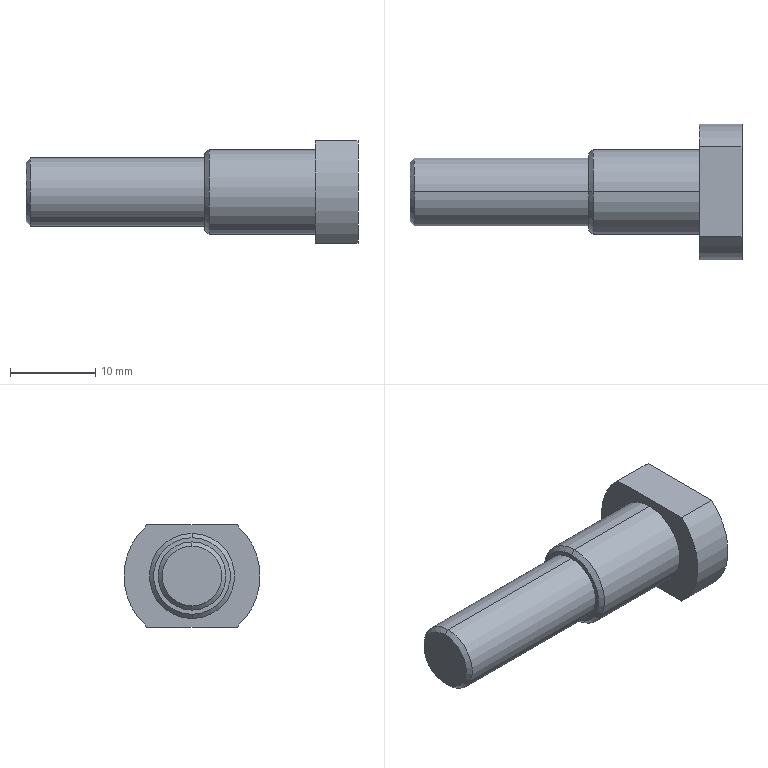Component | SolidWorks | ZTDJ-L-400-04-16-MaterialPortBagClamp-Axis4-2 | 1 solid | 16 faces | box 39 x 16 x 12 mm | volume 2930 mm3 | cylinder 6 | plane 6 | cone 4 | commonest cylinder face diameters 8 x2 10 x2 16 x2 | material 1023 Carbon Steel Sheet (SS)
STEP:
#1=COLOUR_RGB('',0.7922,0.8196,0.9333);
#2=FILL_AREA_STYLE_COLOUR('',#1);
#3=FILL_AREA_STYLE('',(#2));
#4=SURFACE_STYLE_FILL_AREA(#3);
#5=SURFACE_SIDE_STYLE('',(#4));
#6=SURFACE_STYLE_USAGE(.BOTH.,#5);
#7=PRESENTATION_STYLE_ASSIGNMENT((#6));
#8=CARTESIAN_POINT('',(2.365,-0.401,10.492));
#9=VERTEX_POINT('',#8);
#10=CARTESIAN_POINT('',(2.365,-0.401,10.217));
#11=VERTEX_POINT('',#10);
#12=CARTESIAN_POINT('',(2.365,-0.401,10.354));
#13=DIRECTION('',(-1.,0.,0.));
#14=DIRECTION('',(0.,0.,1.));
#15=AXIS2_PLACEMENT_3D('',#12,#13,#14);
#16=CIRCLE('',#15,0.1378);
#17=EDGE_CURVE('',#9,#11,#16,.T.);
#18=ORIENTED_EDGE('',*,*,#17,.F.);
#19=CARTESIAN_POINT('',(2.384,-0.401,10.512));
#20=VERTEX_POINT('',#19);
#21=CARTESIAN_POINT('',(2.365,-0.401,10.492));
#22=DIRECTION('',(0.7071,0.,0.7071));
#23=VECTOR('',#22,39.37);
#24=LINE('',#21,#23);
#25=EDGE_CURVE('',#9,#20,#24,.T.);
#26=ORIENTED_EDGE('',*,*,#25,.T.);
#27=CARTESIAN_POINT('',(2.384,-0.401,10.197));
#28=VERTEX_POINT('',#27);
#29=CARTESIAN_POINT('',(2.384,-0.401,10.354));
#30=DIRECTION('',(1.,0.,0.));
#31=DIRECTION('',(0.,0.,1.));
#32=AXIS2_PLACEMENT_3D('',#29,#30,#31);
#33=CIRCLE('',#32,0.1575);
#34=EDGE_CURVE('',#28,#20,#33,.T.);
#35=ORIENTED_EDGE('',*,*,#34,.F.);
#36=CARTESIAN_POINT('',(2.365,-0.401,10.217));
#37=DIRECTION('',(0.7071,0.,-0.7071));
#38=VECTOR('',#37,39.37);
#39=LINE('',#36,#38);
#40=EDGE_CURVE('',#11,#28,#39,.T.);
#41=ORIENTED_EDGE('',*,*,#40,.F.);
#42=EDGE_LOOP('',(#18,#26,#35,#41));
#43=FACE_OUTER_BOUND('',#42,.T.);
#44=CARTESIAN_POINT('',(2.365,-0.401,10.354));
#45=DIRECTION('',(1.,0.,0.));
#46=DIRECTION('',(0.,0.,-1.));
#47=AXIS2_PLACEMENT_3D('',#44,#45,#46);
#48=CONICAL_SURFACE('',#47,0.1378,0.7854);
#49=ADVANCED_FACE('',(#43),#48,.T.);
#50=ORIENTED_EDGE('',*,*,#34,.T.);
#51=CARTESIAN_POINT('',(3.191,-0.401,10.512));
#52=VERTEX_POINT('',#51);
#53=CARTESIAN_POINT('',(2.365,-0.401,10.512));
#54=DIRECTION('',(1.,0.,0.));
#55=VECTOR('',#54,39.37);
#56=LINE('',#53,#55);
#57=EDGE_CURVE('',#20,#52,#56,.T.);
#58=ORIENTED_EDGE('',*,*,#57,.T.);
#59=CARTESIAN_POINT('',(3.191,-0.401,10.197));
#60=VERTEX_POINT('',#59);
#61=CARTESIAN_POINT('',(3.191,-0.401,10.354));
#62=DIRECTION('',(-1.,0.,0.));
#63=DIRECTION('',(0.,0.,-1.));
#64=AXIS2_PLACEMENT_3D('',#61,#62,#63);
#65=CIRCLE('',#64,0.1575);
#66=EDGE_CURVE('',#52,#60,#65,.T.);
#67=ORIENTED_EDGE('',*,*,#66,.T.);
#68=CARTESIAN_POINT('',(2.365,-0.401,10.197));
#69=DIRECTION('',(1.,0.,0.));
#70=VECTOR('',#69,39.37);
#71=LINE('',#68,#70);
#72=EDGE_CURVE('',#28,#60,#71,.T.);
#73=ORIENTED_EDGE('',*,*,#72,.F.);
#74=EDGE_LOOP('',(#50,#58,#67,#73));
#75=FACE_OUTER_BOUND('',#74,.T.);
#76=CARTESIAN_POINT('',(2.365,-0.401,10.354));
#77=DIRECTION('',(1.,0.,0.));
#78=DIRECTION('',(0.,0.,-1.));
#79=AXIS2_PLACEMENT_3D('',#76,#77,#78);
#80=CYLINDRICAL_SURFACE('',#79,0.1575);
#81=ADVANCED_FACE('',(#75),#80,.T.);
#82=CARTESIAN_POINT('',(3.191,-0.401,10.531));
#83=VERTEX_POINT('',#82);
#84=CARTESIAN_POINT('',(3.191,-0.401,10.177));
#85=VERTEX_POINT('',#84);
#86=CARTESIAN_POINT('',(3.191,-0.401,10.354));
#87=DIRECTION('',(-1.,0.,0.));
#88=DIRECTION('',(0.,0.,-1.));
#89=AXIS2_PLACEMENT_3D('',#86,#87,#88);
#90=CIRCLE('',#89,0.1772);
#91=EDGE_CURVE('',#83,#85,#90,.T.);
#92=ORIENTED_EDGE('',*,*,#91,.F.);
#93=CARTESIAN_POINT('',(3.211,-0.401,10.551));
#94=VERTEX_POINT('',#93);
#95=CARTESIAN_POINT('',(3.211,-0.401,10.551));
#96=DIRECTION('',(0.7071,0.,0.7071));
#97=VECTOR('',#96,39.37);
#98=LINE('',#95,#97);
#99=EDGE_CURVE('',#83,#94,#98,.T.);
#100=ORIENTED_EDGE('',*,*,#99,.T.);
#101=CARTESIAN_POINT('',(3.211,-0.401,10.157));
#102=VERTEX_POINT('',#101);
#103=CARTESIAN_POINT('',(3.211,-0.401,10.354));
#104=DIRECTION('',(1.,0.,0.));
#105=DIRECTION('',(0.,0.,-1.));
#106=AXIS2_PLACEMENT_3D('',#103,#104,#105);
#107=CIRCLE('',#106,0.1969);
#108=EDGE_CURVE('',#102,#94,#107,.T.);
#109=ORIENTED_EDGE('',*,*,#108,.F.);
#110=CARTESIAN_POINT('',(3.211,-0.401,10.157));
#111=DIRECTION('',(0.7071,0.,-0.7071));
#112=VECTOR('',#111,39.37);
#113=LINE('',#110,#112);
#114=EDGE_CURVE('',#85,#102,#113,.T.);
#115=ORIENTED_EDGE('',*,*,#114,.F.);
#116=EDGE_LOOP('',(#92,#100,#109,#115));
#117=FACE_OUTER_BOUND('',#116,.T.);
#118=CARTESIAN_POINT('',(3.211,-0.401,10.354));
#119=DIRECTION('',(1.,0.,0.));
#120=DIRECTION('',(0.,0.,-1.));
#121=AXIS2_PLACEMENT_3D('',#118,#119,#120);
#122=CONICAL_SURFACE('',#121,0.1969,0.7854);
#123=ADVANCED_FACE('',(#117),#122,.T.);
#124=CARTESIAN_POINT('',(3.703,-0.401,10.157));
#125=VERTEX_POINT('',#124);
#126=CARTESIAN_POINT('',(3.703,-0.401,10.551));
#127=VERTEX_POINT('',#126);
#128=CARTESIAN_POINT('',(3.703,-0.401,10.354));
#129=DIRECTION('',(1.,0.,0.));
#130=DIRECTION('',(0.,0.,-1.));
#131=AXIS2_PLACEMENT_3D('',#128,#129,#130);
#132=CIRCLE('',#131,0.1969);
#133=EDGE_CURVE('',#125,#127,#132,.T.);
#134=ORIENTED_EDGE('',*,*,#133,.F.);
#135=CARTESIAN_POINT('',(3.703,-0.401,10.157));
#136=DIRECTION('',(-1.,0.,0.));
#137=VECTOR('',#136,39.37);
#138=LINE('',#135,#137);
#139=EDGE_CURVE('',#125,#102,#138,.T.);
#140=ORIENTED_EDGE('',*,*,#139,.T.);
#141=ORIENTED_EDGE('',*,*,#108,.T.);
#142=CARTESIAN_POINT('',(3.703,-0.401,10.551));
#143=DIRECTION('',(-1.,0.,0.));
#144=VECTOR('',#143,39.37);
#145=LINE('',#142,#144);
#146=EDGE_CURVE('',#127,#94,#145,.T.);
#147=ORIENTED_EDGE('',*,*,#146,.F.);
#148=EDGE_LOOP('',(#134,#140,#141,#147));
#149=FACE_OUTER_BOUND('',#148,.T.);
#150=CARTESIAN_POINT('',(3.703,-0.401,10.354));
#151=DIRECTION('',(-1.,0.,0.));
#152=DIRECTION('',(0.,0.,1.));
#153=AXIS2_PLACEMENT_3D('',#150,#151,#152);
#154=CYLINDRICAL_SURFACE('',#153,0.1969);
#155=ADVANCED_FACE('',(#149),#154,.T.);
#156=CARTESIAN_POINT('',(3.9,-0.6093,10.591));
#157=VERTEX_POINT('',#156);
#158=CARTESIAN_POINT('',(3.9,-0.6093,10.118));
#159=VERTEX_POINT('',#158);
#160=CARTESIAN_POINT('',(3.9,-0.401,10.354));
#161=DIRECTION('',(1.,0.,0.));
#162=DIRECTION('',(0.,0.,-1.));
#163=AXIS2_PLACEMENT_3D('',#160,#161,#162);
#164=CIRCLE('',#163,0.315);
#165=EDGE_CURVE('',#157,#159,#164,.T.);
#166=ORIENTED_EDGE('',*,*,#165,.F.);
#167=CARTESIAN_POINT('',(3.703,-0.6093,10.591));
#168=VERTEX_POINT('',#167);
#169=CARTESIAN_POINT('',(4.136,-0.6093,10.591));
#170=DIRECTION('',(-1.,0.,0.));
#171=VECTOR('',#170,39.37);
#172=LINE('',#169,#171);
#173=EDGE_CURVE('',#157,#168,#172,.T.);
#174=ORIENTED_EDGE('',*,*,#173,.T.);
#175=CARTESIAN_POINT('',(3.703,-0.6093,10.118));
#176=VERTEX_POINT('',#175);
#177=CARTESIAN_POINT('',(3.703,-0.401,10.354));
#178=DIRECTION('',(1.,0.,0.));
#179=DIRECTION('',(0.,0.,-1.));
#180=AXIS2_PLACEMENT_3D('',#177,#178,#179);
#181=CIRCLE('',#180,0.315);
#182=EDGE_CURVE('',#168,#176,#181,.T.);
#183=ORIENTED_EDGE('',*,*,#182,.T.);
#184=CARTESIAN_POINT('',(4.136,-0.6093,10.118));
#185=DIRECTION('',(-1.,0.,0.));
#186=VECTOR('',#185,39.37);
#187=LINE('',#184,#186);
#188=EDGE_CURVE('',#159,#176,#187,.T.);
#189=ORIENTED_EDGE('',*,*,#188,.F.);
#190=EDGE_LOOP('',(#166,#174,#183,#189));
#191=FACE_OUTER_BOUND('',#190,.T.);
#192=CARTESIAN_POINT('',(3.9,-0.401,10.354));
#193=DIRECTION('',(-1.,0.,0.));
#194=DIRECTION('',(0.,0.,1.));
#195=AXIS2_PLACEMENT_3D('',#192,#193,#194);
#196=CYLINDRICAL_SURFACE('',#195,0.315);
#197=ADVANCED_FACE('',(#191),#196,.T.);
#198=CARTESIAN_POINT('',(3.703,-0.401,10.354));
#199=DIRECTION('',(1.,0.,0.));
#200=DIRECTION('',(0.,0.,-1.));
#201=AXIS2_PLACEMENT_3D('',#198,#199,#200);
#202=CIRCLE('',#201,0.1969);
#203=EDGE_CURVE('',#127,#125,#202,.T.);
#204=ORIENTED_EDGE('',*,*,#203,.T.);
#205=ORIENTED_EDGE('',*,*,#133,.T.);
#206=EDGE_LOOP('',(#204,#205));
#207=FACE_BOUND('',#206,.T.);
#208=ORIENTED_EDGE('',*,*,#182,.F.);
#209=CARTESIAN_POINT('',(3.703,-0.1927,10.591));
#210=VERTEX_POINT('',#209);
#211=CARTESIAN_POINT('',(3.703,-0.401,10.591));
#212=DIRECTION('',(0.,-1.,0.));
#213=VECTOR('',#212,39.37);
#214=LINE('',#211,#213);
#215=EDGE_CURVE('',#210,#168,#214,.T.);
#216=ORIENTED_EDGE('',*,*,#215,.F.);
#217=CARTESIAN_POINT('',(3.703,-0.1927,10.118));
#218=VERTEX_POINT('',#217);
#219=CARTESIAN_POINT('',(3.703,-0.401,10.354));
#220=DIRECTION('',(1.,0.,0.));
#221=DIRECTION('',(0.,0.,-1.));
#222=AXIS2_PLACEMENT_3D('',#219,#220,#221);
#223=CIRCLE('',#222,0.315);
#224=EDGE_CURVE('',#218,#210,#223,.T.);
#225=ORIENTED_EDGE('',*,*,#224,.F.);
#226=CARTESIAN_POINT('',(3.703,-0.401,10.118));
#227=DIRECTION('',(0.,-1.,0.));
#228=VECTOR('',#227,39.37);
#229=LINE('',#226,#228);
#230=EDGE_CURVE('',#218,#176,#229,.T.);
#231=ORIENTED_EDGE('',*,*,#230,.T.);
#232=EDGE_LOOP('',(#208,#216,#225,#231));
#233=FACE_OUTER_BOUND('',#232,.T.);
#234=CARTESIAN_POINT('',(3.703,-0.401,10.354));
#235=DIRECTION('',(1.,0.,0.));
#236=DIRECTION('',(0.,0.,-1.));
#237=AXIS2_PLACEMENT_3D('',#234,#235,#236);
#238=PLANE('',#237);
#239=ADVANCED_FACE('',(#207,#233),#238,.F.);
#240=ORIENTED_EDGE('',*,*,#224,.T.);
#241=CARTESIAN_POINT('',(3.9,-0.1927,10.591));
#242=VERTEX_POINT('',#241);
#243=CARTESIAN_POINT('',(4.136,-0.1927,10.591));
#244=DIRECTION('',(-1.,0.,0.));
#245=VECTOR('',#244,39.37);
#246=LINE('',#243,#245);
#247=EDGE_CURVE('',#242,#210,#246,.T.);
#248=ORIENTED_EDGE('',*,*,#247,.F.);
#249=CARTESIAN_POINT('',(3.9,-0.1927,10.118));
#250=VERTEX_POINT('',#249);
#251=CARTESIAN_POINT('',(3.9,-0.401,10.354));
#252=DIRECTION('',(1.,0.,0.));
#253=DIRECTION('',(0.,0.,-1.));
#254=AXIS2_PLACEMENT_3D('',#251,#252,#253);
#255=CIRCLE('',#254,0.315);
#256=EDGE_CURVE('',#250,#242,#255,.T.);
#257=ORIENTED_EDGE('',*,*,#256,.F.);
#258=CARTESIAN_POINT('',(4.136,-0.1927,10.118));
#259=DIRECTION('',(-1.,0.,0.));
#260=VECTOR('',#259,39.37);
#261=LINE('',#258,#260);
#262=EDGE_CURVE('',#250,#218,#261,.T.);
#263=ORIENTED_EDGE('',*,*,#262,.T.);
#264=EDGE_LOOP('',(#240,#248,#257,#263));
#265=FACE_OUTER_BOUND('',#264,.T.);
#266=CARTESIAN_POINT('',(3.9,-0.401,10.354));
#267=DIRECTION('',(-1.,0.,0.));
#268=DIRECTION('',(0.,0.,1.));
#269=AXIS2_PLACEMENT_3D('',#266,#267,#268);
#270=CYLINDRICAL_SURFACE('',#269,0.315);
#271=ADVANCED_FACE('',(#265),#270,.T.);
#272=CARTESIAN_POINT('',(3.9,-0.401,10.591));
#273=DIRECTION('',(0.,1.,0.));
#274=VECTOR('',#273,39.37);
#275=LINE('',#272,#274);
#276=EDGE_CURVE('',#157,#242,#275,.T.);
#277=ORIENTED_EDGE('',*,*,#276,.F.);
#278=ORIENTED_EDGE('',*,*,#165,.T.);
#279=CARTESIAN_POINT('',(3.9,-0.401,10.118));
#280=DIRECTION('',(0.,1.,0.));
#281=VECTOR('',#280,39.37);
#282=LINE('',#279,#281);
#283=EDGE_CURVE('',#159,#250,#282,.T.);
#284=ORIENTED_EDGE('',*,*,#283,.T.);
#285=ORIENTED_EDGE('',*,*,#256,.T.);
#286=EDGE_LOOP('',(#277,#278,#284,#285));
#287=FACE_OUTER_BOUND('',#286,.T.);
#288=CARTESIAN_POINT('',(3.9,-0.401,10.354));
#289=DIRECTION('',(1.,0.,0.));
#290=DIRECTION('',(0.,0.,-1.));
#291=AXIS2_PLACEMENT_3D('',#288,#289,#290);
#292=PLANE('',#291);
#293=ADVANCED_FACE('',(#287),#292,.T.);
#294=CARTESIAN_POINT('',(3.191,-0.401,10.354));
#295=DIRECTION('',(-1.,0.,0.));
#296=DIRECTION('',(0.,0.,-1.));
#297=AXIS2_PLACEMENT_3D('',#294,#295,#296);
#298=CIRCLE('',#297,0.1772);
#299=EDGE_CURVE('',#85,#83,#298,.T.);
#300=ORIENTED_EDGE('',*,*,#299,.T.);
#301=ORIENTED_EDGE('',*,*,#91,.T.);
#302=EDGE_LOOP('',(#300,#301));
#303=FACE_OUTER_BOUND('',#302,.T.);
#304=CARTESIAN_POINT('',(3.191,-0.401,10.354));
#305=DIRECTION('',(-1.,0.,0.));
#306=DIRECTION('',(0.,0.,-1.));
#307=AXIS2_PLACEMENT_3D('',#304,#305,#306);
#308=CIRCLE('',#307,0.1575);
#309=EDGE_CURVE('',#60,#52,#308,.T.);
#310=ORIENTED_EDGE('',*,*,#309,.F.);
#311=ORIENTED_EDGE('',*,*,#66,.F.);
#312=EDGE_LOOP('',(#310,#311));
#313=FACE_BOUND('',#312,.T.);
#314=CARTESIAN_POINT('',(3.191,-0.401,10.354));
#315=DIRECTION('',(1.,0.,0.));
#316=DIRECTION('',(0.,0.,-1.));
#317=AXIS2_PLACEMENT_3D('',#314,#315,#316);
#318=PLANE('',#317);
#319=ADVANCED_FACE('',(#303,#313),#318,.F.);
#320=ORIENTED_EDGE('',*,*,#139,.F.);
#321=ORIENTED_EDGE('',*,*,#203,.F.);
#322=ORIENTED_EDGE('',*,*,#146,.T.);
#323=CARTESIAN_POINT('',(3.211,-0.401,10.354));
#324=DIRECTION('',(1.,0.,0.));
#325=DIRECTION('',(0.,0.,-1.));
#326=AXIS2_PLACEMENT_3D('',#323,#324,#325);
#327=CIRCLE('',#326,0.1969);
#328=EDGE_CURVE('',#94,#102,#327,.T.);
#329=ORIENTED_EDGE('',*,*,#328,.T.);
#330=EDGE_LOOP('',(#320,#321,#322,#329));
#331=FACE_OUTER_BOUND('',#330,.T.);
#332=CARTESIAN_POINT('',(3.703,-0.401,10.354));
#333=DIRECTION('',(-1.,0.,0.));
#334=DIRECTION('',(0.,0.,1.));
#335=AXIS2_PLACEMENT_3D('',#332,#333,#334);
#336=CYLINDRICAL_SURFACE('',#335,0.1969);
#337=ADVANCED_FACE('',(#331),#336,.T.);
#338=ORIENTED_EDGE('',*,*,#99,.F.);
#339=ORIENTED_EDGE('',*,*,#299,.F.);
#340=ORIENTED_EDGE('',*,*,#114,.T.);
#341=ORIENTED_EDGE('',*,*,#328,.F.);
#342=EDGE_LOOP('',(#338,#339,#340,#341));
#343=FACE_OUTER_BOUND('',#342,.T.);
#344=CARTESIAN_POINT('',(3.211,-0.401,10.354));
#345=DIRECTION('',(1.,0.,0.));
#346=DIRECTION('',(0.,0.,-1.));
#347=AXIS2_PLACEMENT_3D('',#344,#345,#346);
#348=CONICAL_SURFACE('',#347,0.1969,0.7854);
#349=ADVANCED_FACE('',(#343),#348,.T.);
#350=ORIENTED_EDGE('',*,*,#57,.F.);
#351=CARTESIAN_POINT('',(2.384,-0.401,10.354));
#352=DIRECTION('',(1.,0.,0.));
#353=DIRECTION('',(0.,0.,1.));
#354=AXIS2_PLACEMENT_3D('',#351,#352,#353);
#355=CIRCLE('',#354,0.1575);
#356=EDGE_CURVE('',#20,#28,#355,.T.);
#357=ORIENTED_EDGE('',*,*,#356,.T.);
#358=ORIENTED_EDGE('',*,*,#72,.T.);
#359=ORIENTED_EDGE('',*,*,#309,.T.);
#360=EDGE_LOOP('',(#350,#357,#358,#359));
#361=FACE_OUTER_BOUND('',#360,.T.);
#362=CARTESIAN_POINT('',(2.365,-0.401,10.354));
#363=DIRECTION('',(1.,0.,0.));
#364=DIRECTION('',(0.,0.,-1.));
#365=AXIS2_PLACEMENT_3D('',#362,#363,#364);
#366=CYLINDRICAL_SURFACE('',#365,0.1575);
#367=ADVANCED_FACE('',(#361),#366,.T.);
#368=CARTESIAN_POINT('',(2.365,-0.401,10.354));
#369=DIRECTION('',(-1.,0.,0.));
#370=DIRECTION('',(0.,0.,1.));
#371=AXIS2_PLACEMENT_3D('',#368,#369,#370);
#372=CIRCLE('',#371,0.1378);
#373=EDGE_CURVE('',#11,#9,#372,.T.);
#374=ORIENTED_EDGE('',*,*,#373,.T.);
#375=ORIENTED_EDGE('',*,*,#17,.T.);
#376=EDGE_LOOP('',(#374,#375));
#377=FACE_OUTER_BOUND('',#376,.T.);
#378=CARTESIAN_POINT('',(2.365,-0.401,10.354));
#379=DIRECTION('',(-1.,0.,0.));
#380=DIRECTION('',(0.,0.,1.));
#381=AXIS2_PLACEMENT_3D('',#378,#379,#380);
#382=PLANE('',#381);
#383=ADVANCED_FACE('',(#377),#382,.T.);
#384=ORIENTED_EDGE('',*,*,#25,.F.);
#385=ORIENTED_EDGE('',*,*,#373,.F.);
#386=ORIENTED_EDGE('',*,*,#40,.T.);
#387=ORIENTED_EDGE('',*,*,#356,.F.);
#388=EDGE_LOOP('',(#384,#385,#386,#387));
#389=FACE_OUTER_BOUND('',#388,.T.);
#390=CARTESIAN_POINT('',(2.365,-0.401,10.354));
#391=DIRECTION('',(1.,0.,0.));
#392=DIRECTION('',(0.,0.,-1.));
#393=AXIS2_PLACEMENT_3D('',#390,#391,#392);
#394=CONICAL_SURFACE('',#393,0.1378,0.7854);
#395=ADVANCED_FACE('',(#389),#394,.T.);
#396=ORIENTED_EDGE('',*,*,#188,.T.);
#397=ORIENTED_EDGE('',*,*,#230,.F.);
#398=ORIENTED_EDGE('',*,*,#262,.F.);
#399=ORIENTED_EDGE('',*,*,#283,.F.);
#400=EDGE_LOOP('',(#396,#397,#398,#399));
#401=FACE_OUTER_BOUND('',#400,.T.);
#402=CARTESIAN_POINT('',(4.136,-0.401,10.118));
#403=DIRECTION('',(0.,0.,-1.));
#404=DIRECTION('',(-1.,0.,0.));
#405=AXIS2_PLACEMENT_3D('',#402,#403,#404);
#406=PLANE('',#405);
#407=ADVANCED_FACE('',(#401),#406,.T.);
#408=ORIENTED_EDGE('',*,*,#276,.T.);
#409=ORIENTED_EDGE('',*,*,#247,.T.);
#410=ORIENTED_EDGE('',*,*,#215,.T.);
#411=ORIENTED_EDGE('',*,*,#173,.F.);
#412=EDGE_LOOP('',(#408,#409,#410,#411));
#413=FACE_OUTER_BOUND('',#412,.T.);
#414=CARTESIAN_POINT('',(4.136,-0.401,10.591));
#415=DIRECTION('',(0.,0.,-1.));
#416=DIRECTION('',(-1.,0.,0.));
#417=AXIS2_PLACEMENT_3D('',#414,#415,#416);
#418=PLANE('',#417);
#419=ADVANCED_FACE('',(#413),#418,.F.);
#420=CLOSED_SHELL('',(#49,#81,#123,#155,#197,#239,#271,#293,#319,#337,#349,#367,#383,#395,#407,#419));
#421=MANIFOLD_SOLID_BREP('',#420);
#422=STYLED_ITEM('',(#7),#421);
#423=PRESENTATION_LAYER_ASSIGNMENT('','',(#422));
#424=CARTESIAN_POINT('',(0.,0.,0.));
#425=DIRECTION('',(0.,0.,1.));
#426=DIRECTION('',(1.,0.,0.));
#427=AXIS2_PLACEMENT_3D('',#424,#425,#426);
#428=(LENGTH_UNIT()NAMED_UNIT(*)SI_UNIT($,.METRE.));
#429=LENGTH_MEASURE_WITH_UNIT(LENGTH_MEASURE(0.0254),#428);
#430=DIMENSIONAL_EXPONENTS(1.,0.,0.,0.,0.,0.,0.);
#431=(CONVERSION_BASED_UNIT('',#429)LENGTH_UNIT()NAMED_UNIT(#430));
#432=UNCERTAINTY_MEASURE_WITH_UNIT(LENGTH_MEASURE(0.00001),#431,'','');
#433=(NAMED_UNIT(*)PLANE_ANGLE_UNIT()SI_UNIT($,.RADIAN.));
#434=(NAMED_UNIT(*)SI_UNIT($,.STERADIAN.)SOLID_ANGLE_UNIT());
#435=(GEOMETRIC_REPRESENTATION_CONTEXT(3)GLOBAL_UNCERTAINTY_ASSIGNED_CONTEXT((#432))GLOBAL_UNIT_ASSIGNED_CONTEXT((#431,#433,#434))REPRESENTATION_CONTEXT('',''));
#436=ADVANCED_BREP_SHAPE_REPRESENTATION('',(#421,#427),#435);
#437=(LENGTH_UNIT()NAMED_UNIT(*)SI_UNIT($,.METRE.));
#438=LENGTH_MEASURE_WITH_UNIT(LENGTH_MEASURE(0.0254),#437);
#439=DIMENSIONAL_EXPONENTS(1.,0.,0.,0.,0.,0.,0.);
#440=(CONVERSION_BASED_UNIT('',#438)LENGTH_UNIT()NAMED_UNIT(#439));
#441=UNCERTAINTY_MEASURE_WITH_UNIT(LENGTH_MEASURE(0.00001),#440,'','');
#442=(NAMED_UNIT(*)PLANE_ANGLE_UNIT()SI_UNIT($,.RADIAN.));
#443=(NAMED_UNIT(*)SI_UNIT($,.STERADIAN.)SOLID_ANGLE_UNIT());
#444=(GEOMETRIC_REPRESENTATION_CONTEXT(3)GLOBAL_UNCERTAINTY_ASSIGNED_CONTEXT((#441))GLOBAL_UNIT_ASSIGNED_CONTEXT((#440,#442,#443))REPRESENTATION_CONTEXT('',''));
#445=MECHANICAL_DESIGN_GEOMETRIC_PRESENTATION_REPRESENTATION('',(#422),#444);